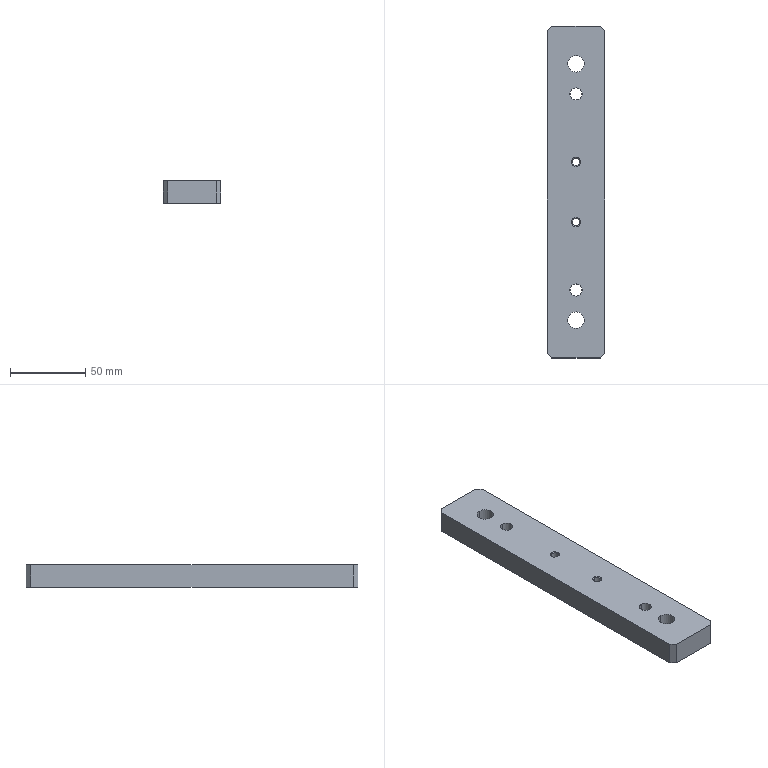Component | SolidWorks | DirectPressureVerticalSeal-1_TransitionPlate-1 | 1 solid | 30 faces | box 38 x 220 x 15 mm | volume 120177 mm3 | cylinder 12 | plane 10 | cone 8 | commonest cylinder face diameters 5 x4 8 x4 11 x4
build123d program:
from build123d import *

# Parameters (mm, degrees)
BOSS_EXTRUDE1_DEPTH                                  = 15
F_11_0_11_DIAMETER_HOLE1_D                           = 11
CONICAL_COUNTERSUNK_HOLE_1_FOR_M6_FLAT_H_D           = 8
CONICAL_COUNTERSUNK_HOLE_1_FOR_M6_FLAT_H_CSINK_D     = 8.05
CONICAL_COUNTERSUNK_HOLE_1_FOR_M6_FLAT_H_CSINK_ANGLE = 90
F_5_0_5_DIAMETER_HOLE1_D                             = 5
F_5_0_5_DIAMETER_HOLE1_CSINK_D                       = 6.05
F_5_0_5_DIAMETER_HOLE1_CSINK_ANGLE                   = 90


with BuildPart() as part:
    # Sketch1 → Boss-Extrude1 (new body)
    with BuildSketch(Plane.XY.offset(7.5)):
        Polygon((-110, 16), (-110, -16), (-107, -19), (107, -19), (110, -16), (110, 16), (107, 19), (-107, 19), align=None)
    extrude(amount=-BOSS_EXTRUDE1_DEPTH)

    # 11.0 _11_ Diameter Hole1 (through all)
    with Locations(Plane(origin=(0, 0, -7.5), x_dir=(-1, 0, 0), z_dir=(0, 0, -1))):
        with Locations((-85, 0), (85, 0)):
            Hole(F_11_0_11_DIAMETER_HOLE1_D / 2)

    # Conical Countersunk Hole 1 for M6 Flat H (through all)
    with Locations(Plane.XY.offset(7.5)):
        with Locations((65, 0), (-65, 0)):
            CounterSinkHole(CONICAL_COUNTERSUNK_HOLE_1_FOR_M6_FLAT_H_D / 2, CONICAL_COUNTERSUNK_HOLE_1_FOR_M6_FLAT_H_CSINK_D / 2, counter_sink_angle=CONICAL_COUNTERSUNK_HOLE_1_FOR_M6_FLAT_H_CSINK_ANGLE)

    # 5.0 _5_ Diameter Hole1 (through all)
    with Locations(Plane.XY.offset(7.5)):
        with Locations((20, 0), (-20, 0)):
            CounterSinkHole(F_5_0_5_DIAMETER_HOLE1_D / 2, F_5_0_5_DIAMETER_HOLE1_CSINK_D / 2, counter_sink_angle=F_5_0_5_DIAMETER_HOLE1_CSINK_ANGLE)


solid = part.part

# Placed as in the assembly
solid = solid.moved(Location((-298.746, 246.873, 246.554), (0, 0, 90)))
STEP:
#1=COLOUR_RGB('',0.7922,0.8196,0.9333);
#2=FILL_AREA_STYLE_COLOUR('',#1);
#3=FILL_AREA_STYLE('',(#2));
#4=SURFACE_STYLE_FILL_AREA(#3);
#5=SURFACE_SIDE_STYLE('',(#4));
#6=SURFACE_STYLE_USAGE(.BOTH.,#5);
#7=PRESENTATION_STYLE_ASSIGNMENT((#6));
#8=CARTESIAN_POINT('',(-11.762,9.03,9.981));
#9=VERTEX_POINT('',#8);
#10=CARTESIAN_POINT('',(-11.762,8.834,9.981));
#11=VERTEX_POINT('',#10);
#12=CARTESIAN_POINT('',(-11.762,8.932,9.981));
#13=DIRECTION('',(-0.,0.,1.));
#14=DIRECTION('',(0.,-1.,0.));
#15=AXIS2_PLACEMENT_3D('',#12,#13,#14);
#16=CIRCLE('',#15,0.09843);
#17=EDGE_CURVE('',#9,#11,#16,.T.);
#18=ORIENTED_EDGE('',*,*,#17,.F.);
#19=CARTESIAN_POINT('',(-11.762,9.051,10.002));
#20=VERTEX_POINT('',#19);
#21=CARTESIAN_POINT('',(-11.762,9.051,10.002));
#22=DIRECTION('',(0.,0.7071,0.7071));
#23=VECTOR('',#22,39.37);
#24=LINE('',#21,#23);
#25=EDGE_CURVE('',#9,#20,#24,.T.);
#26=ORIENTED_EDGE('',*,*,#25,.T.);
#27=CARTESIAN_POINT('',(-11.762,8.813,10.002));
#28=VERTEX_POINT('',#27);
#29=CARTESIAN_POINT('',(-11.762,8.932,10.002));
#30=DIRECTION('',(-0.,0.,1.));
#31=DIRECTION('',(0.,-1.,0.));
#32=AXIS2_PLACEMENT_3D('',#29,#30,#31);
#33=CIRCLE('',#32,0.1191);
#34=EDGE_CURVE('',#20,#28,#33,.T.);
#35=ORIENTED_EDGE('',*,*,#34,.T.);
#36=CARTESIAN_POINT('',(-11.762,8.813,10.002));
#37=DIRECTION('',(-0.,-0.7071,0.7071));
#38=VECTOR('',#37,39.37);
#39=LINE('',#36,#38);
#40=EDGE_CURVE('',#11,#28,#39,.T.);
#41=ORIENTED_EDGE('',*,*,#40,.F.);
#42=EDGE_LOOP('',(#18,#26,#35,#41));
#43=FACE_OUTER_BOUND('',#42,.T.);
#44=CARTESIAN_POINT('',(-11.762,8.932,10.002));
#45=DIRECTION('',(-0.,0.,1.));
#46=DIRECTION('',(0.,-1.,0.));
#47=AXIS2_PLACEMENT_3D('',#44,#45,#46);
#48=CONICAL_SURFACE('',#47,0.1191,0.7854);
#49=ADVANCED_FACE('',(#43),#48,.F.);
#50=CARTESIAN_POINT('',(-11.762,9.03,9.412));
#51=VERTEX_POINT('',#50);
#52=CARTESIAN_POINT('',(-11.762,8.834,9.412));
#53=VERTEX_POINT('',#52);
#54=CARTESIAN_POINT('',(-11.762,8.932,9.412));
#55=DIRECTION('',(-0.,0.,1.));
#56=DIRECTION('',(0.,-1.,0.));
#57=AXIS2_PLACEMENT_3D('',#54,#55,#56);
#58=CIRCLE('',#57,0.09843);
#59=EDGE_CURVE('',#51,#53,#58,.T.);
#60=ORIENTED_EDGE('',*,*,#59,.F.);
#61=CARTESIAN_POINT('',(-11.762,9.03,10.002));
#62=DIRECTION('',(-0.,0.,1.));
#63=VECTOR('',#62,39.37);
#64=LINE('',#61,#63);
#65=EDGE_CURVE('',#51,#9,#64,.T.);
#66=ORIENTED_EDGE('',*,*,#65,.T.);
#67=ORIENTED_EDGE('',*,*,#17,.T.);
#68=CARTESIAN_POINT('',(-11.762,8.834,10.002));
#69=DIRECTION('',(-0.,0.,1.));
#70=VECTOR('',#69,39.37);
#71=LINE('',#68,#70);
#72=EDGE_CURVE('',#53,#11,#71,.T.);
#73=ORIENTED_EDGE('',*,*,#72,.F.);
#74=EDGE_LOOP('',(#60,#66,#67,#73));
#75=FACE_OUTER_BOUND('',#74,.T.);
#76=CARTESIAN_POINT('',(-11.762,8.932,10.002));
#77=DIRECTION('',(-0.,0.,1.));
#78=DIRECTION('',(0.,-1.,0.));
#79=AXIS2_PLACEMENT_3D('',#76,#77,#78);
#80=CYLINDRICAL_SURFACE('',#79,0.09843);
#81=ADVANCED_FACE('',(#75),#80,.F.);
#82=CARTESIAN_POINT('',(-11.762,10.605,9.981));
#83=VERTEX_POINT('',#82);
#84=CARTESIAN_POINT('',(-11.762,10.408,9.981));
#85=VERTEX_POINT('',#84);
#86=CARTESIAN_POINT('',(-11.762,10.507,9.981));
#87=DIRECTION('',(-0.,0.,1.));
#88=DIRECTION('',(0.,-1.,0.));
#89=AXIS2_PLACEMENT_3D('',#86,#87,#88);
#90=CIRCLE('',#89,0.09843);
#91=EDGE_CURVE('',#83,#85,#90,.T.);
#92=ORIENTED_EDGE('',*,*,#91,.F.);
#93=CARTESIAN_POINT('',(-11.762,10.626,10.002));
#94=VERTEX_POINT('',#93);
#95=CARTESIAN_POINT('',(-11.762,10.626,10.002));
#96=DIRECTION('',(0.,0.7071,0.7071));
#97=VECTOR('',#96,39.37);
#98=LINE('',#95,#97);
#99=EDGE_CURVE('',#83,#94,#98,.T.);
#100=ORIENTED_EDGE('',*,*,#99,.T.);
#101=CARTESIAN_POINT('',(-11.762,10.388,10.002));
#102=VERTEX_POINT('',#101);
#103=CARTESIAN_POINT('',(-11.762,10.507,10.002));
#104=DIRECTION('',(-0.,0.,1.));
#105=DIRECTION('',(0.,-1.,0.));
#106=AXIS2_PLACEMENT_3D('',#103,#104,#105);
#107=CIRCLE('',#106,0.1191);
#108=EDGE_CURVE('',#94,#102,#107,.T.);
#109=ORIENTED_EDGE('',*,*,#108,.T.);
#110=CARTESIAN_POINT('',(-11.762,10.388,10.002));
#111=DIRECTION('',(-0.,-0.7071,0.7071));
#112=VECTOR('',#111,39.37);
#113=LINE('',#110,#112);
#114=EDGE_CURVE('',#85,#102,#113,.T.);
#115=ORIENTED_EDGE('',*,*,#114,.F.);
#116=EDGE_LOOP('',(#92,#100,#109,#115));
#117=FACE_OUTER_BOUND('',#116,.T.);
#118=CARTESIAN_POINT('',(-11.762,10.507,10.002));
#119=DIRECTION('',(-0.,0.,1.));
#120=DIRECTION('',(0.,-1.,0.));
#121=AXIS2_PLACEMENT_3D('',#118,#119,#120);
#122=CONICAL_SURFACE('',#121,0.1191,0.7854);
#123=ADVANCED_FACE('',(#117),#122,.F.);
#124=CARTESIAN_POINT('',(-11.762,10.605,9.412));
#125=VERTEX_POINT('',#124);
#126=CARTESIAN_POINT('',(-11.762,10.408,9.412));
#127=VERTEX_POINT('',#126);
#128=CARTESIAN_POINT('',(-11.762,10.507,9.412));
#129=DIRECTION('',(-0.,0.,1.));
#130=DIRECTION('',(0.,-1.,0.));
#131=AXIS2_PLACEMENT_3D('',#128,#129,#130);
#132=CIRCLE('',#131,0.09843);
#133=EDGE_CURVE('',#125,#127,#132,.T.);
#134=ORIENTED_EDGE('',*,*,#133,.F.);
#135=CARTESIAN_POINT('',(-11.762,10.605,10.002));
#136=DIRECTION('',(-0.,0.,1.));
#137=VECTOR('',#136,39.37);
#138=LINE('',#135,#137);
#139=EDGE_CURVE('',#125,#83,#138,.T.);
#140=ORIENTED_EDGE('',*,*,#139,.T.);
#141=ORIENTED_EDGE('',*,*,#91,.T.);
#142=CARTESIAN_POINT('',(-11.762,10.408,10.002));
#143=DIRECTION('',(-0.,0.,1.));
#144=VECTOR('',#143,39.37);
#145=LINE('',#142,#144);
#146=EDGE_CURVE('',#127,#85,#145,.T.);
#147=ORIENTED_EDGE('',*,*,#146,.F.);
#148=EDGE_LOOP('',(#134,#140,#141,#147));
#149=FACE_OUTER_BOUND('',#148,.T.);
#150=CARTESIAN_POINT('',(-11.762,10.507,10.002));
#151=DIRECTION('',(-0.,0.,1.));
#152=DIRECTION('',(0.,-1.,0.));
#153=AXIS2_PLACEMENT_3D('',#150,#151,#152);
#154=CYLINDRICAL_SURFACE('',#153,0.09843);
#155=ADVANCED_FACE('',(#149),#154,.F.);
#156=CARTESIAN_POINT('',(-11.762,7.318,10.001));
#157=VERTEX_POINT('',#156);
#158=CARTESIAN_POINT('',(-11.762,7.003,10.001));
#159=VERTEX_POINT('',#158);
#160=CARTESIAN_POINT('',(-11.762,7.16,10.001));
#161=DIRECTION('',(-0.,0.,1.));
#162=DIRECTION('',(0.,-1.,0.));
#163=AXIS2_PLACEMENT_3D('',#160,#161,#162);
#164=CIRCLE('',#163,0.1575);
#165=EDGE_CURVE('',#157,#159,#164,.T.);
#166=ORIENTED_EDGE('',*,*,#165,.F.);
#167=CARTESIAN_POINT('',(-11.762,7.319,10.002));
#168=VERTEX_POINT('',#167);
#169=CARTESIAN_POINT('',(-11.762,7.319,10.002));
#170=DIRECTION('',(0.,0.7071,0.7071));
#171=VECTOR('',#170,39.37);
#172=LINE('',#169,#171);
#173=EDGE_CURVE('',#157,#168,#172,.T.);
#174=ORIENTED_EDGE('',*,*,#173,.T.);
#175=CARTESIAN_POINT('',(-11.762,7.002,10.002));
#176=VERTEX_POINT('',#175);
#177=CARTESIAN_POINT('',(-11.762,7.16,10.002));
#178=DIRECTION('',(-0.,0.,1.));
#179=DIRECTION('',(0.,-1.,0.));
#180=AXIS2_PLACEMENT_3D('',#177,#178,#179);
#181=CIRCLE('',#180,0.1585);
#182=EDGE_CURVE('',#168,#176,#181,.T.);
#183=ORIENTED_EDGE('',*,*,#182,.T.);
#184=CARTESIAN_POINT('',(-11.762,7.002,10.002));
#185=DIRECTION('',(-0.,-0.7071,0.7071));
#186=VECTOR('',#185,39.37);
#187=LINE('',#184,#186);
#188=EDGE_CURVE('',#159,#176,#187,.T.);
#189=ORIENTED_EDGE('',*,*,#188,.F.);
#190=EDGE_LOOP('',(#166,#174,#183,#189));
#191=FACE_OUTER_BOUND('',#190,.T.);
#192=CARTESIAN_POINT('',(-11.762,7.16,10.002));
#193=DIRECTION('',(-0.,0.,1.));
#194=DIRECTION('',(0.,-1.,0.));
#195=AXIS2_PLACEMENT_3D('',#192,#193,#194);
#196=CONICAL_SURFACE('',#195,0.1585,0.7854);
#197=ADVANCED_FACE('',(#191),#196,.F.);
#198=CARTESIAN_POINT('',(-11.762,7.318,9.412));
#199=VERTEX_POINT('',#198);
#200=CARTESIAN_POINT('',(-11.762,7.003,9.412));
#201=VERTEX_POINT('',#200);
#202=CARTESIAN_POINT('',(-11.762,7.16,9.412));
#203=DIRECTION('',(-0.,0.,1.));
#204=DIRECTION('',(0.,-1.,0.));
#205=AXIS2_PLACEMENT_3D('',#202,#203,#204);
#206=CIRCLE('',#205,0.1575);
#207=EDGE_CURVE('',#199,#201,#206,.T.);
#208=ORIENTED_EDGE('',*,*,#207,.F.);
#209=CARTESIAN_POINT('',(-11.762,7.318,10.002));
#210=DIRECTION('',(-0.,0.,1.));
#211=VECTOR('',#210,39.37);
#212=LINE('',#209,#211);
#213=EDGE_CURVE('',#199,#157,#212,.T.);
#214=ORIENTED_EDGE('',*,*,#213,.T.);
#215=ORIENTED_EDGE('',*,*,#165,.T.);
#216=CARTESIAN_POINT('',(-11.762,7.003,10.002));
#217=DIRECTION('',(-0.,0.,1.));
#218=VECTOR('',#217,39.37);
#219=LINE('',#216,#218);
#220=EDGE_CURVE('',#201,#159,#219,.T.);
#221=ORIENTED_EDGE('',*,*,#220,.F.);
#222=EDGE_LOOP('',(#208,#214,#215,#221));
#223=FACE_OUTER_BOUND('',#222,.T.);
#224=CARTESIAN_POINT('',(-11.762,7.16,10.002));
#225=DIRECTION('',(-0.,0.,1.));
#226=DIRECTION('',(0.,-1.,0.));
#227=AXIS2_PLACEMENT_3D('',#224,#225,#226);
#228=CYLINDRICAL_SURFACE('',#227,0.1575);
#229=ADVANCED_FACE('',(#223),#228,.F.);
#230=CARTESIAN_POINT('',(-11.762,12.436,10.001));
#231=VERTEX_POINT('',#230);
#232=CARTESIAN_POINT('',(-11.762,12.121,10.001));
#233=VERTEX_POINT('',#232);
#234=CARTESIAN_POINT('',(-11.762,12.278,10.001));
#235=DIRECTION('',(-0.,0.,1.));
#236=DIRECTION('',(0.,-1.,0.));
#237=AXIS2_PLACEMENT_3D('',#234,#235,#236);
#238=CIRCLE('',#237,0.1575);
#239=EDGE_CURVE('',#231,#233,#238,.T.);
#240=ORIENTED_EDGE('',*,*,#239,.F.);
#241=CARTESIAN_POINT('',(-11.762,12.437,10.002));
#242=VERTEX_POINT('',#241);
#243=CARTESIAN_POINT('',(-11.762,12.437,10.002));
#244=DIRECTION('',(0.,0.7071,0.7071));
#245=VECTOR('',#244,39.37);
#246=LINE('',#243,#245);
#247=EDGE_CURVE('',#231,#242,#246,.T.);
#248=ORIENTED_EDGE('',*,*,#247,.T.);
#249=CARTESIAN_POINT('',(-11.762,12.12,10.002));
#250=VERTEX_POINT('',#249);
#251=CARTESIAN_POINT('',(-11.762,12.278,10.002));
#252=DIRECTION('',(-0.,0.,1.));
#253=DIRECTION('',(0.,-1.,0.));
#254=AXIS2_PLACEMENT_3D('',#251,#252,#253);
#255=CIRCLE('',#254,0.1585);
#256=EDGE_CURVE('',#242,#250,#255,.T.);
#257=ORIENTED_EDGE('',*,*,#256,.T.);
#258=CARTESIAN_POINT('',(-11.762,12.12,10.002));
#259=DIRECTION('',(-0.,-0.7071,0.7071));
#260=VECTOR('',#259,39.37);
#261=LINE('',#258,#260);
#262=EDGE_CURVE('',#233,#250,#261,.T.);
#263=ORIENTED_EDGE('',*,*,#262,.F.);
#264=EDGE_LOOP('',(#240,#248,#257,#263));
#265=FACE_OUTER_BOUND('',#264,.T.);
#266=CARTESIAN_POINT('',(-11.762,12.278,10.002));
#267=DIRECTION('',(-0.,0.,1.));
#268=DIRECTION('',(0.,-1.,0.));
#269=AXIS2_PLACEMENT_3D('',#266,#267,#268);
#270=CONICAL_SURFACE('',#269,0.1585,0.7854);
#271=ADVANCED_FACE('',(#265),#270,.F.);
#272=CARTESIAN_POINT('',(-11.762,12.436,9.412));
#273=VERTEX_POINT('',#272);
#274=CARTESIAN_POINT('',(-11.762,12.121,9.412));
#275=VERTEX_POINT('',#274);
#276=CARTESIAN_POINT('',(-11.762,12.278,9.412));
#277=DIRECTION('',(-0.,0.,1.));
#278=DIRECTION('',(0.,-1.,0.));
#279=AXIS2_PLACEMENT_3D('',#276,#277,#278);
#280=CIRCLE('',#279,0.1575);
#281=EDGE_CURVE('',#273,#275,#280,.T.);
#282=ORIENTED_EDGE('',*,*,#281,.F.);
#283=CARTESIAN_POINT('',(-11.762,12.436,10.002));
#284=DIRECTION('',(-0.,0.,1.));
#285=VECTOR('',#284,39.37);
#286=LINE('',#283,#285);
#287=EDGE_CURVE('',#273,#231,#286,.T.);
#288=ORIENTED_EDGE('',*,*,#287,.T.);
#289=ORIENTED_EDGE('',*,*,#239,.T.);
#290=CARTESIAN_POINT('',(-11.762,12.121,10.002));
#291=DIRECTION('',(-0.,0.,1.));
#292=VECTOR('',#291,39.37);
#293=LINE('',#290,#292);
#294=EDGE_CURVE('',#275,#233,#293,.T.);
#295=ORIENTED_EDGE('',*,*,#294,.F.);
#296=EDGE_LOOP('',(#282,#288,#289,#295));
#297=FACE_OUTER_BOUND('',#296,.T.);
#298=CARTESIAN_POINT('',(-11.762,12.278,10.002));
#299=DIRECTION('',(-0.,0.,1.));
#300=DIRECTION('',(0.,-1.,0.));
#301=AXIS2_PLACEMENT_3D('',#298,#299,#300);
#302=CYLINDRICAL_SURFACE('',#301,0.1575);
#303=ADVANCED_FACE('',(#297),#302,.F.);
#304=CARTESIAN_POINT('',(-11.762,6.156,10.002));
#305=VERTEX_POINT('',#304);
#306=CARTESIAN_POINT('',(-11.762,6.59,10.002));
#307=VERTEX_POINT('',#306);
#308=CARTESIAN_POINT('',(-11.762,6.373,10.002));
#309=DIRECTION('',(0.,-0.,-1.));
#310=DIRECTION('',(0.,1.,0.));
#311=AXIS2_PLACEMENT_3D('',#308,#309,#310);
#312=CIRCLE('',#311,0.2165);
#313=EDGE_CURVE('',#305,#307,#312,.T.);
#314=ORIENTED_EDGE('',*,*,#313,.F.);
#315=CARTESIAN_POINT('',(-11.762,6.156,9.412));
#316=VERTEX_POINT('',#315);
#317=CARTESIAN_POINT('',(-11.762,6.156,9.412));
#318=DIRECTION('',(0.,-0.,-1.));
#319=VECTOR('',#318,39.37);
#320=LINE('',#317,#319);
#321=EDGE_CURVE('',#305,#316,#320,.T.);
#322=ORIENTED_EDGE('',*,*,#321,.T.);
#323=CARTESIAN_POINT('',(-11.762,6.59,9.412));
#324=VERTEX_POINT('',#323);
#325=CARTESIAN_POINT('',(-11.762,6.373,9.412));
#326=DIRECTION('',(0.,-0.,-1.));
#327=DIRECTION('',(0.,1.,0.));
#328=AXIS2_PLACEMENT_3D('',#325,#326,#327);
#329=CIRCLE('',#328,0.2165);
#330=EDGE_CURVE('',#316,#324,#329,.T.);
#331=ORIENTED_EDGE('',*,*,#330,.T.);
#332=CARTESIAN_POINT('',(-11.762,6.59,9.412));
#333=DIRECTION('',(0.,-0.,-1.));
#334=VECTOR('',#333,39.37);
#335=LINE('',#332,#334);
#336=EDGE_CURVE('',#307,#324,#335,.T.);
#337=ORIENTED_EDGE('',*,*,#336,.F.);
#338=EDGE_LOOP('',(#314,#322,#331,#337));
#339=FACE_OUTER_BOUND('',#338,.T.);
#340=CARTESIAN_POINT('',(-11.762,6.373,9.412));
#341=DIRECTION('',(0.,-0.,-1.));
#342=DIRECTION('',(0.,1.,0.));
#343=AXIS2_PLACEMENT_3D('',#340,#341,#342);
#344=CYLINDRICAL_SURFACE('',#343,0.2165);
#345=ADVANCED_FACE('',(#339),#344,.F.);
#346=CARTESIAN_POINT('',(-11.762,12.849,10.002));
#347=VERTEX_POINT('',#346);
#348=CARTESIAN_POINT('',(-11.762,13.282,10.002));
#349=VERTEX_POINT('',#348);
#350=CARTESIAN_POINT('',(-11.762,13.066,10.002));
#351=DIRECTION('',(0.,-0.,-1.));
#352=DIRECTION('',(0.,1.,0.));
#353=AXIS2_PLACEMENT_3D('',#350,#351,#352);
#354=CIRCLE('',#353,0.2165);
#355=EDGE_CURVE('',#347,#349,#354,.T.);
#356=ORIENTED_EDGE('',*,*,#355,.F.);
#357=CARTESIAN_POINT('',(-11.762,12.849,9.412));
#358=VERTEX_POINT('',#357);
#359=CARTESIAN_POINT('',(-11.762,12.849,9.412));
#360=DIRECTION('',(0.,-0.,-1.));
#361=VECTOR('',#360,39.37);
#362=LINE('',#359,#361);
#363=EDGE_CURVE('',#347,#358,#362,.T.);
#364=ORIENTED_EDGE('',*,*,#363,.T.);
#365=CARTESIAN_POINT('',(-11.762,13.282,9.412));
#366=VERTEX_POINT('',#365);
#367=CARTESIAN_POINT('',(-11.762,13.066,9.412));
#368=DIRECTION('',(0.,-0.,-1.));
#369=DIRECTION('',(0.,1.,0.));
#370=AXIS2_PLACEMENT_3D('',#367,#368,#369);
#371=CIRCLE('',#370,0.2165);
#372=EDGE_CURVE('',#358,#366,#371,.T.);
#373=ORIENTED_EDGE('',*,*,#372,.T.);
#374=CARTESIAN_POINT('',(-11.762,13.282,9.412));
#375=DIRECTION('',(0.,-0.,-1.));
#376=VECTOR('',#375,39.37);
#377=LINE('',#374,#376);
#378=EDGE_CURVE('',#349,#366,#377,.T.);
#379=ORIENTED_EDGE('',*,*,#378,.F.);
#380=EDGE_LOOP('',(#356,#364,#373,#379));
#381=FACE_OUTER_BOUND('',#380,.T.);
#382=CARTESIAN_POINT('',(-11.762,13.066,9.412));
#383=DIRECTION('',(0.,-0.,-1.));
#384=DIRECTION('',(0.,1.,0.));
#385=AXIS2_PLACEMENT_3D('',#382,#383,#384);
#386=CYLINDRICAL_SURFACE('',#385,0.2165);
#387=ADVANCED_FACE('',(#381),#386,.F.);
#388=CARTESIAN_POINT('',(-11.014,13.932,10.002));
#389=VERTEX_POINT('',#388);
#390=CARTESIAN_POINT('',(-11.132,14.05,10.002));
#391=VERTEX_POINT('',#390);
#392=CARTESIAN_POINT('',(-11.014,13.932,10.002));
#393=DIRECTION('',(-0.7071,0.7071,-0.));
#394=VECTOR('',#393,39.37);
#395=LINE('',#392,#394);
#396=EDGE_CURVE('',#389,#391,#395,.T.);
#397=ORIENTED_EDGE('',*,*,#396,.F.);
#398=CARTESIAN_POINT('',(-11.014,13.932,9.412));
#399=VERTEX_POINT('',#398);
#400=CARTESIAN_POINT('',(-11.014,13.932,9.412));
#401=DIRECTION('',(-0.,0.,1.));
#402=VECTOR('',#401,39.37);
#403=LINE('',#400,#402);
#404=EDGE_CURVE('',#399,#389,#403,.T.);
#405=ORIENTED_EDGE('',*,*,#404,.F.);
#406=CARTESIAN_POINT('',(-11.132,14.05,9.412));
#407=VERTEX_POINT('',#406);
#408=CARTESIAN_POINT('',(-11.014,13.932,9.412));
#409=DIRECTION('',(-0.7071,0.7071,-0.));
#410=VECTOR('',#409,39.37);
#411=LINE('',#408,#410);
#412=EDGE_CURVE('',#399,#407,#411,.T.);
#413=ORIENTED_EDGE('',*,*,#412,.T.);
#414=CARTESIAN_POINT('',(-11.132,14.05,9.412));
#415=DIRECTION('',(-0.,0.,1.));
#416=VECTOR('',#415,39.37);
#417=LINE('',#414,#416);
#418=EDGE_CURVE('',#407,#391,#417,.T.);
#419=ORIENTED_EDGE('',*,*,#418,.T.);
#420=EDGE_LOOP('',(#397,#405,#413,#419));
#421=FACE_OUTER_BOUND('',#420,.T.);
#422=CARTESIAN_POINT('',(-11.014,13.932,9.412));
#423=DIRECTION('',(0.7071,0.7071,0.));
#424=DIRECTION('',(-0.7071,0.7071,-0.));
#425=AXIS2_PLACEMENT_3D('',#422,#423,#424);
#426=PLANE('',#425);
#427=ADVANCED_FACE('',(#421),#426,.T.);
#428=CARTESIAN_POINT('',(-11.014,5.507,10.002));
#429=VERTEX_POINT('',#428);
#430=CARTESIAN_POINT('',(-11.014,5.507,10.002));
#431=DIRECTION('',(0.,1.,-0.));
#432=VECTOR('',#431,39.37);
#433=LINE('',#430,#432);
#434=EDGE_CURVE('',#429,#389,#433,.T.);
#435=ORIENTED_EDGE('',*,*,#434,.F.);
#436=CARTESIAN_POINT('',(-11.014,5.507,9.412));
#437=VERTEX_POINT('',#436);
#438=CARTESIAN_POINT('',(-11.014,5.507,9.412));
#439=DIRECTION('',(-0.,0.,1.));
#440=VECTOR('',#439,39.37);
#441=LINE('',#438,#440);
#442=EDGE_CURVE('',#437,#429,#441,.T.);
#443=ORIENTED_EDGE('',*,*,#442,.F.);
#444=CARTESIAN_POINT('',(-11.014,5.507,9.412));
#445=DIRECTION('',(0.,1.,-0.));
#446=VECTOR('',#445,39.37);
#447=LINE('',#444,#446);
#448=EDGE_CURVE('',#437,#399,#447,.T.);
#449=ORIENTED_EDGE('',*,*,#448,.T.);
#450=ORIENTED_EDGE('',*,*,#404,.T.);
#451=EDGE_LOOP('',(#435,#443,#449,#450));
#452=FACE_OUTER_BOUND('',#451,.T.);
#453=CARTESIAN_POINT('',(-11.014,5.507,9.412));
#454=DIRECTION('',(1.,-0.,0.));
#455=DIRECTION('',(-0.,0.,1.));
#456=AXIS2_PLACEMENT_3D('',#453,#454,#455);
#457=PLANE('',#456);
#458=ADVANCED_FACE('',(#452),#457,.T.);
#459=CARTESIAN_POINT('',(-11.132,5.389,10.002));
#460=VERTEX_POINT('',#459);
#461=CARTESIAN_POINT('',(-11.132,5.389,10.002));
#462=DIRECTION('',(0.7071,0.7071,0.));
#463=VECTOR('',#462,39.37);
#464=LINE('',#461,#463);
#465=EDGE_CURVE('',#460,#429,#464,.T.);
#466=ORIENTED_EDGE('',*,*,#465,.F.);
#467=CARTESIAN_POINT('',(-11.132,5.389,9.412));
#468=VERTEX_POINT('',#467);
#469=CARTESIAN_POINT('',(-11.132,5.389,9.412));
#470=DIRECTION('',(-0.,0.,1.));
#471=VECTOR('',#470,39.37);
#472=LINE('',#469,#471);
#473=EDGE_CURVE('',#468,#460,#472,.T.);
#474=ORIENTED_EDGE('',*,*,#473,.F.);
#475=CARTESIAN_POINT('',(-11.132,5.389,9.412));
#476=DIRECTION('',(0.7071,0.7071,0.));
#477=VECTOR('',#476,39.37);
#478=LINE('',#475,#477);
#479=EDGE_CURVE('',#468,#437,#478,.T.);
#480=ORIENTED_EDGE('',*,*,#479,.T.);
#481=ORIENTED_EDGE('',*,*,#442,.T.);
#482=EDGE_LOOP('',(#466,#474,#480,#481));
#483=FACE_OUTER_BOUND('',#482,.T.);
#484=CARTESIAN_POINT('',(-11.132,5.389,9.412));
#485=DIRECTION('',(0.7071,-0.7071,0.));
#486=DIRECTION('',(0.7071,0.7071,0.));
#487=AXIS2_PLACEMENT_3D('',#484,#485,#486);
#488=PLANE('',#487);
#489=ADVANCED_FACE('',(#483),#488,.T.);
#490=CARTESIAN_POINT('',(-12.392,5.389,10.002));
#491=VERTEX_POINT('',#490);
#492=CARTESIAN_POINT('',(-12.392,5.389,10.002));
#493=DIRECTION('',(1.,-0.,0.));
#494=VECTOR('',#493,39.37);
#495=LINE('',#492,#494);
#496=EDGE_CURVE('',#491,#460,#495,.T.);
#497=ORIENTED_EDGE('',*,*,#496,.F.);
#498=CARTESIAN_POINT('',(-12.392,5.389,9.412));
#499=VERTEX_POINT('',#498);
#500=CARTESIAN_POINT('',(-12.392,5.389,9.412));
#501=DIRECTION('',(-0.,0.,1.));
#502=VECTOR('',#501,39.37);
#503=LINE('',#500,#502);
#504=EDGE_CURVE('',#499,#491,#503,.T.);
#505=ORIENTED_EDGE('',*,*,#504,.F.);
#506=CARTESIAN_POINT('',(-12.392,5.389,9.412));
#507=DIRECTION('',(1.,-0.,0.));
#508=VECTOR('',#507,39.37);
#509=LINE('',#506,#508);
#510=EDGE_CURVE('',#499,#468,#509,.T.);
#511=ORIENTED_EDGE('',*,*,#510,.T.);
#512=ORIENTED_EDGE('',*,*,#473,.T.);
#513=EDGE_LOOP('',(#497,#505,#511,#512));
#514=FACE_OUTER_BOUND('',#513,.T.);
#515=CARTESIAN_POINT('',(-12.392,5.389,9.412));
#516=DIRECTION('',(-0.,-1.,0.));
#517=DIRECTION('',(0.,-0.,-1.));
#518=AXIS2_PLACEMENT_3D('',#515,#516,#517);
#519=PLANE('',#518);
#520=ADVANCED_FACE('',(#514),#519,.T.);
#521=CARTESIAN_POINT('',(-12.51,5.507,10.002));
#522=VERTEX_POINT('',#521);
#523=CARTESIAN_POINT('',(-12.51,5.507,10.002));
#524=DIRECTION('',(0.7071,-0.7071,0.));
#525=VECTOR('',#524,39.37);
#526=LINE('',#523,#525);
#527=EDGE_CURVE('',#522,#491,#526,.T.);
#528=ORIENTED_EDGE('',*,*,#527,.F.);
#529=CARTESIAN_POINT('',(-12.51,5.507,9.412));
#530=VERTEX_POINT('',#529);
#531=CARTESIAN_POINT('',(-12.51,5.507,9.412));
#532=DIRECTION('',(-0.,0.,1.));
#533=VECTOR('',#532,39.37);
#534=LINE('',#531,#533);
#535=EDGE_CURVE('',#530,#522,#534,.T.);
#536=ORIENTED_EDGE('',*,*,#535,.F.);
#537=CARTESIAN_POINT('',(-12.51,5.507,9.412));
#538=DIRECTION('',(0.7071,-0.7071,0.));
#539=VECTOR('',#538,39.37);
#540=LINE('',#537,#539);
#541=EDGE_CURVE('',#530,#499,#540,.T.);
#542=ORIENTED_EDGE('',*,*,#541,.T.);
#543=ORIENTED_EDGE('',*,*,#504,.T.);
#544=EDGE_LOOP('',(#528,#536,#542,#543));
#545=FACE_OUTER_BOUND('',#544,.T.);
#546=CARTESIAN_POINT('',(-12.51,5.507,9.412));
#547=DIRECTION('',(-0.7071,-0.7071,-0.));
#548=DIRECTION('',(0.7071,-0.7071,0.));
#549=AXIS2_PLACEMENT_3D('',#546,#547,#548);
#550=PLANE('',#549);
#551=ADVANCED_FACE('',(#545),#550,.T.);
#552=CARTESIAN_POINT('',(-12.51,13.932,10.002));
#553=VERTEX_POINT('',#552);
#554=CARTESIAN_POINT('',(-12.51,13.932,10.002));
#555=DIRECTION('',(-0.,-1.,0.));
#556=VECTOR('',#555,39.37);
#557=LINE('',#554,#556);
#558=EDGE_CURVE('',#553,#522,#557,.T.);
#559=ORIENTED_EDGE('',*,*,#558,.F.);
#560=CARTESIAN_POINT('',(-12.51,13.932,9.412));
#561=VERTEX_POINT('',#560);
#562=CARTESIAN_POINT('',(-12.51,13.932,9.412));
#563=DIRECTION('',(-0.,0.,1.));
#564=VECTOR('',#563,39.37);
#565=LINE('',#562,#564);
#566=EDGE_CURVE('',#561,#553,#565,.T.);
#567=ORIENTED_EDGE('',*,*,#566,.F.);
#568=CARTESIAN_POINT('',(-12.51,13.932,9.412));
#569=DIRECTION('',(-0.,-1.,0.));
#570=VECTOR('',#569,39.37);
#571=LINE('',#568,#570);
#572=EDGE_CURVE('',#561,#530,#571,.T.);
#573=ORIENTED_EDGE('',*,*,#572,.T.);
#574=ORIENTED_EDGE('',*,*,#535,.T.);
#575=EDGE_LOOP('',(#559,#567,#573,#574));
#576=FACE_OUTER_BOUND('',#575,.T.);
#577=CARTESIAN_POINT('',(-12.51,13.932,9.412));
#578=DIRECTION('',(-1.,0.,-0.));
#579=DIRECTION('',(0.,-0.,-1.));
#580=AXIS2_PLACEMENT_3D('',#577,#578,#579);
#581=PLANE('',#580);
#582=ADVANCED_FACE('',(#576),#581,.T.);
#583=CARTESIAN_POINT('',(-12.392,14.05,10.002));
#584=VERTEX_POINT('',#583);
#585=CARTESIAN_POINT('',(-12.392,14.05,10.002));
#586=DIRECTION('',(-0.7071,-0.7071,-0.));
#587=VECTOR('',#586,39.37);
#588=LINE('',#585,#587);
#589=EDGE_CURVE('',#584,#553,#588,.T.);
#590=ORIENTED_EDGE('',*,*,#589,.F.);
#591=CARTESIAN_POINT('',(-12.392,14.05,9.412));
#592=VERTEX_POINT('',#591);
#593=CARTESIAN_POINT('',(-12.392,14.05,9.412));
#594=DIRECTION('',(-0.,0.,1.));
#595=VECTOR('',#594,39.37);
#596=LINE('',#593,#595);
#597=EDGE_CURVE('',#592,#584,#596,.T.);
#598=ORIENTED_EDGE('',*,*,#597,.F.);
#599=CARTESIAN_POINT('',(-12.392,14.05,9.412));
#600=DIRECTION('',(-0.7071,-0.7071,-0.));
#601=VECTOR('',#600,39.37);
#602=LINE('',#599,#601);
#603=EDGE_CURVE('',#592,#561,#602,.T.);
#604=ORIENTED_EDGE('',*,*,#603,.T.);
#605=ORIENTED_EDGE('',*,*,#566,.T.);
#606=EDGE_LOOP('',(#590,#598,#604,#605));
#607=FACE_OUTER_BOUND('',#606,.T.);
#608=CARTESIAN_POINT('',(-12.392,14.05,9.412));
#609=DIRECTION('',(-0.7071,0.7071,-0.));
#610=DIRECTION('',(-0.7071,-0.7071,-0.));
#611=AXIS2_PLACEMENT_3D('',#608,#609,#610);
#612=PLANE('',#611);
#613=ADVANCED_FACE('',(#607),#612,.T.);
#614=CARTESIAN_POINT('',(-11.132,14.05,10.002));
#615=DIRECTION('',(-1.,0.,-0.));
#616=VECTOR('',#615,39.37);
#617=LINE('',#614,#616);
#618=EDGE_CURVE('',#391,#584,#617,.T.);
#619=ORIENTED_EDGE('',*,*,#618,.F.);
#620=ORIENTED_EDGE('',*,*,#418,.F.);
#621=CARTESIAN_POINT('',(-11.132,14.05,9.412));
#622=DIRECTION('',(-1.,0.,-0.));
#623=VECTOR('',#622,39.37);
#624=LINE('',#621,#623);
#625=EDGE_CURVE('',#407,#592,#624,.T.);
#626=ORIENTED_EDGE('',*,*,#625,.T.);
#627=ORIENTED_EDGE('',*,*,#597,.T.);
#628=EDGE_LOOP('',(#619,#620,#626,#627));
#629=FACE_OUTER_BOUND('',#628,.T.);
#630=CARTESIAN_POINT('',(-11.132,14.05,9.412));
#631=DIRECTION('',(0.,1.,-0.));
#632=DIRECTION('',(-1.,0.,-0.));
#633=AXIS2_PLACEMENT_3D('',#630,#631,#632);
#634=PLANE('',#633);
#635=ADVANCED_FACE('',(#629),#634,.T.);
#636=CARTESIAN_POINT('',(-11.762,8.932,9.412));
#637=DIRECTION('',(-0.,0.,1.));
#638=DIRECTION('',(0.,-1.,0.));
#639=AXIS2_PLACEMENT_3D('',#636,#637,#638);
#640=CIRCLE('',#639,0.09843);
#641=EDGE_CURVE('',#53,#51,#640,.T.);
#642=ORIENTED_EDGE('',*,*,#641,.T.);
#643=ORIENTED_EDGE('',*,*,#59,.T.);
#644=EDGE_LOOP('',(#642,#643));
#645=FACE_BOUND('',#644,.T.);
#646=CARTESIAN_POINT('',(-11.762,10.507,9.412));
#647=DIRECTION('',(-0.,0.,1.));
#648=DIRECTION('',(0.,-1.,0.));
#649=AXIS2_PLACEMENT_3D('',#646,#647,#648);
#650=CIRCLE('',#649,0.09843);
#651=EDGE_CURVE('',#127,#125,#650,.T.);
#652=ORIENTED_EDGE('',*,*,#651,.T.);
#653=ORIENTED_EDGE('',*,*,#133,.T.);
#654=EDGE_LOOP('',(#652,#653));
#655=FACE_BOUND('',#654,.T.);
#656=CARTESIAN_POINT('',(-11.762,7.16,9.412));
#657=DIRECTION('',(-0.,0.,1.));
#658=DIRECTION('',(0.,-1.,0.));
#659=AXIS2_PLACEMENT_3D('',#656,#657,#658);
#660=CIRCLE('',#659,0.1575);
#661=EDGE_CURVE('',#201,#199,#660,.T.);
#662=ORIENTED_EDGE('',*,*,#661,.T.);
#663=ORIENTED_EDGE('',*,*,#207,.T.);
#664=EDGE_LOOP('',(#662,#663));
#665=FACE_BOUND('',#664,.T.);
#666=CARTESIAN_POINT('',(-11.762,12.278,9.412));
#667=DIRECTION('',(-0.,0.,1.));
#668=DIRECTION('',(0.,-1.,0.));
#669=AXIS2_PLACEMENT_3D('',#666,#667,#668);
#670=CIRCLE('',#669,0.1575);
#671=EDGE_CURVE('',#275,#273,#670,.T.);
#672=ORIENTED_EDGE('',*,*,#671,.T.);
#673=ORIENTED_EDGE('',*,*,#281,.T.);
#674=EDGE_LOOP('',(#672,#673));
#675=FACE_BOUND('',#674,.T.);
#676=CARTESIAN_POINT('',(-11.762,6.373,9.412));
#677=DIRECTION('',(0.,-0.,-1.));
#678=DIRECTION('',(0.,1.,0.));
#679=AXIS2_PLACEMENT_3D('',#676,#677,#678);
#680=CIRCLE('',#679,0.2165);
#681=EDGE_CURVE('',#324,#316,#680,.T.);
#682=ORIENTED_EDGE('',*,*,#681,.F.);
#683=ORIENTED_EDGE('',*,*,#330,.F.);
#684=EDGE_LOOP('',(#682,#683));
#685=FACE_BOUND('',#684,.T.);
#686=CARTESIAN_POINT('',(-11.762,13.066,9.412));
#687=DIRECTION('',(0.,-0.,-1.));
#688=DIRECTION('',(0.,1.,0.));
#689=AXIS2_PLACEMENT_3D('',#686,#687,#688);
#690=CIRCLE('',#689,0.2165);
#691=EDGE_CURVE('',#366,#358,#690,.T.);
#692=ORIENTED_EDGE('',*,*,#691,.F.);
#693=ORIENTED_EDGE('',*,*,#372,.F.);
#694=EDGE_LOOP('',(#692,#693));
#695=FACE_BOUND('',#694,.T.);
#696=ORIENTED_EDGE('',*,*,#412,.F.);
#697=ORIENTED_EDGE('',*,*,#448,.F.);
#698=ORIENTED_EDGE('',*,*,#479,.F.);
#699=ORIENTED_EDGE('',*,*,#510,.F.);
#700=ORIENTED_EDGE('',*,*,#541,.F.);
#701=ORIENTED_EDGE('',*,*,#572,.F.);
#702=ORIENTED_EDGE('',*,*,#603,.F.);
#703=ORIENTED_EDGE('',*,*,#625,.F.);
#704=EDGE_LOOP('',(#696,#697,#698,#699,#700,#701,#702,#703));
#705=FACE_OUTER_BOUND('',#704,.T.);
#706=CARTESIAN_POINT('',(-11.762,9.719,9.412));
#707=DIRECTION('',(-0.,0.,1.));
#708=DIRECTION('',(-0.,-1.,0.));
#709=AXIS2_PLACEMENT_3D('',#706,#707,#708);
#710=PLANE('',#709);
#711=ADVANCED_FACE('',(#645,#655,#665,#675,#685,#695,#705),#710,.F.);
#712=CARTESIAN_POINT('',(-11.762,8.932,10.002));
#713=DIRECTION('',(-0.,0.,1.));
#714=DIRECTION('',(0.,-1.,0.));
#715=AXIS2_PLACEMENT_3D('',#712,#713,#714);
#716=CIRCLE('',#715,0.1191);
#717=EDGE_CURVE('',#28,#20,#716,.T.);
#718=ORIENTED_EDGE('',*,*,#717,.F.);
#719=ORIENTED_EDGE('',*,*,#34,.F.);
#720=EDGE_LOOP('',(#718,#719));
#721=FACE_BOUND('',#720,.T.);
#722=CARTESIAN_POINT('',(-11.762,10.507,10.002));
#723=DIRECTION('',(-0.,0.,1.));
#724=DIRECTION('',(0.,-1.,0.));
#725=AXIS2_PLACEMENT_3D('',#722,#723,#724);
#726=CIRCLE('',#725,0.1191);
#727=EDGE_CURVE('',#102,#94,#726,.T.);
#728=ORIENTED_EDGE('',*,*,#727,.F.);
#729=ORIENTED_EDGE('',*,*,#108,.F.);
#730=EDGE_LOOP('',(#728,#729));
#731=FACE_BOUND('',#730,.T.);
#732=CARTESIAN_POINT('',(-11.762,7.16,10.002));
#733=DIRECTION('',(-0.,0.,1.));
#734=DIRECTION('',(0.,-1.,0.));
#735=AXIS2_PLACEMENT_3D('',#732,#733,#734);
#736=CIRCLE('',#735,0.1585);
#737=EDGE_CURVE('',#176,#168,#736,.T.);
#738=ORIENTED_EDGE('',*,*,#737,.F.);
#739=ORIENTED_EDGE('',*,*,#182,.F.);
#740=EDGE_LOOP('',(#738,#739));
#741=FACE_BOUND('',#740,.T.);
#742=CARTESIAN_POINT('',(-11.762,12.278,10.002));
#743=DIRECTION('',(-0.,0.,1.));
#744=DIRECTION('',(0.,-1.,0.));
#745=AXIS2_PLACEMENT_3D('',#742,#743,#744);
#746=CIRCLE('',#745,0.1585);
#747=EDGE_CURVE('',#250,#242,#746,.T.);
#748=ORIENTED_EDGE('',*,*,#747,.F.);
#749=ORIENTED_EDGE('',*,*,#256,.F.);
#750=EDGE_LOOP('',(#748,#749));
#751=FACE_BOUND('',#750,.T.);
#752=CARTESIAN_POINT('',(-11.762,6.373,10.002));
#753=DIRECTION('',(0.,-0.,-1.));
#754=DIRECTION('',(0.,1.,0.));
#755=AXIS2_PLACEMENT_3D('',#752,#753,#754);
#756=CIRCLE('',#755,0.2165);
#757=EDGE_CURVE('',#307,#305,#756,.T.);
#758=ORIENTED_EDGE('',*,*,#757,.T.);
#759=ORIENTED_EDGE('',*,*,#313,.T.);
#760=EDGE_LOOP('',(#758,#759));
#761=FACE_BOUND('',#760,.T.);
#762=CARTESIAN_POINT('',(-11.762,13.066,10.002));
#763=DIRECTION('',(0.,-0.,-1.));
#764=DIRECTION('',(0.,1.,0.));
#765=AXIS2_PLACEMENT_3D('',#762,#763,#764);
#766=CIRCLE('',#765,0.2165);
#767=EDGE_CURVE('',#349,#347,#766,.T.);
#768=ORIENTED_EDGE('',*,*,#767,.T.);
#769=ORIENTED_EDGE('',*,*,#355,.T.);
#770=EDGE_LOOP('',(#768,#769));
#771=FACE_BOUND('',#770,.T.);
#772=ORIENTED_EDGE('',*,*,#396,.T.);
#773=ORIENTED_EDGE('',*,*,#618,.T.);
#774=ORIENTED_EDGE('',*,*,#589,.T.);
#775=ORIENTED_EDGE('',*,*,#558,.T.);
#776=ORIENTED_EDGE('',*,*,#527,.T.);
#777=ORIENTED_EDGE('',*,*,#496,.T.);
#778=ORIENTED_EDGE('',*,*,#465,.T.);
#779=ORIENTED_EDGE('',*,*,#434,.T.);
#780=EDGE_LOOP('',(#772,#773,#774,#775,#776,#777,#778,#779));
#781=FACE_OUTER_BOUND('',#780,.T.);
#782=CARTESIAN_POINT('',(-11.762,9.719,10.002));
#783=DIRECTION('',(-0.,0.,1.));
#784=DIRECTION('',(-0.,-1.,0.));
#785=AXIS2_PLACEMENT_3D('',#782,#783,#784);
#786=PLANE('',#785);
#787=ADVANCED_FACE('',(#721,#731,#741,#751,#761,#771,#781),#786,.T.);
#788=ORIENTED_EDGE('',*,*,#363,.F.);
#789=ORIENTED_EDGE('',*,*,#767,.F.);
#790=ORIENTED_EDGE('',*,*,#378,.T.);
#791=ORIENTED_EDGE('',*,*,#691,.T.);
#792=EDGE_LOOP('',(#788,#789,#790,#791));
#793=FACE_OUTER_BOUND('',#792,.T.);
#794=CARTESIAN_POINT('',(-11.762,13.066,9.412));
#795=DIRECTION('',(0.,-0.,-1.));
#796=DIRECTION('',(0.,1.,0.));
#797=AXIS2_PLACEMENT_3D('',#794,#795,#796);
#798=CYLINDRICAL_SURFACE('',#797,0.2165);
#799=ADVANCED_FACE('',(#793),#798,.F.);
#800=ORIENTED_EDGE('',*,*,#321,.F.);
#801=ORIENTED_EDGE('',*,*,#757,.F.);
#802=ORIENTED_EDGE('',*,*,#336,.T.);
#803=ORIENTED_EDGE('',*,*,#681,.T.);
#804=EDGE_LOOP('',(#800,#801,#802,#803));
#805=FACE_OUTER_BOUND('',#804,.T.);
#806=CARTESIAN_POINT('',(-11.762,6.373,9.412));
#807=DIRECTION('',(0.,-0.,-1.));
#808=DIRECTION('',(0.,1.,0.));
#809=AXIS2_PLACEMENT_3D('',#806,#807,#808);
#810=CYLINDRICAL_SURFACE('',#809,0.2165);
#811=ADVANCED_FACE('',(#805),#810,.F.);
#812=ORIENTED_EDGE('',*,*,#287,.F.);
#813=ORIENTED_EDGE('',*,*,#671,.F.);
#814=ORIENTED_EDGE('',*,*,#294,.T.);
#815=CARTESIAN_POINT('',(-11.762,12.278,10.001));
#816=DIRECTION('',(-0.,0.,1.));
#817=DIRECTION('',(0.,-1.,0.));
#818=AXIS2_PLACEMENT_3D('',#815,#816,#817);
#819=CIRCLE('',#818,0.1575);
#820=EDGE_CURVE('',#233,#231,#819,.T.);
#821=ORIENTED_EDGE('',*,*,#820,.T.);
#822=EDGE_LOOP('',(#812,#813,#814,#821));
#823=FACE_OUTER_BOUND('',#822,.T.);
#824=CARTESIAN_POINT('',(-11.762,12.278,10.002));
#825=DIRECTION('',(-0.,0.,1.));
#826=DIRECTION('',(0.,-1.,0.));
#827=AXIS2_PLACEMENT_3D('',#824,#825,#826);
#828=CYLINDRICAL_SURFACE('',#827,0.1575);
#829=ADVANCED_FACE('',(#823),#828,.F.);
#830=ORIENTED_EDGE('',*,*,#247,.F.);
#831=ORIENTED_EDGE('',*,*,#820,.F.);
#832=ORIENTED_EDGE('',*,*,#262,.T.);
#833=ORIENTED_EDGE('',*,*,#747,.T.);
#834=EDGE_LOOP('',(#830,#831,#832,#833));
#835=FACE_OUTER_BOUND('',#834,.T.);
#836=CARTESIAN_POINT('',(-11.762,12.278,10.002));
#837=DIRECTION('',(-0.,0.,1.));
#838=DIRECTION('',(0.,-1.,0.));
#839=AXIS2_PLACEMENT_3D('',#836,#837,#838);
#840=CONICAL_SURFACE('',#839,0.1585,0.7854);
#841=ADVANCED_FACE('',(#835),#840,.F.);
#842=ORIENTED_EDGE('',*,*,#213,.F.);
#843=ORIENTED_EDGE('',*,*,#661,.F.);
#844=ORIENTED_EDGE('',*,*,#220,.T.);
#845=CARTESIAN_POINT('',(-11.762,7.16,10.001));
#846=DIRECTION('',(-0.,0.,1.));
#847=DIRECTION('',(0.,-1.,0.));
#848=AXIS2_PLACEMENT_3D('',#845,#846,#847);
#849=CIRCLE('',#848,0.1575);
#850=EDGE_CURVE('',#159,#157,#849,.T.);
#851=ORIENTED_EDGE('',*,*,#850,.T.);
#852=EDGE_LOOP('',(#842,#843,#844,#851));
#853=FACE_OUTER_BOUND('',#852,.T.);
#854=CARTESIAN_POINT('',(-11.762,7.16,10.002));
#855=DIRECTION('',(-0.,0.,1.));
#856=DIRECTION('',(0.,-1.,0.));
#857=AXIS2_PLACEMENT_3D('',#854,#855,#856);
#858=CYLINDRICAL_SURFACE('',#857,0.1575);
#859=ADVANCED_FACE('',(#853),#858,.F.);
#860=ORIENTED_EDGE('',*,*,#173,.F.);
#861=ORIENTED_EDGE('',*,*,#850,.F.);
#862=ORIENTED_EDGE('',*,*,#188,.T.);
#863=ORIENTED_EDGE('',*,*,#737,.T.);
#864=EDGE_LOOP('',(#860,#861,#862,#863));
#865=FACE_OUTER_BOUND('',#864,.T.);
#866=CARTESIAN_POINT('',(-11.762,7.16,10.002));
#867=DIRECTION('',(-0.,0.,1.));
#868=DIRECTION('',(0.,-1.,0.));
#869=AXIS2_PLACEMENT_3D('',#866,#867,#868);
#870=CONICAL_SURFACE('',#869,0.1585,0.7854);
#871=ADVANCED_FACE('',(#865),#870,.F.);
#872=ORIENTED_EDGE('',*,*,#139,.F.);
#873=ORIENTED_EDGE('',*,*,#651,.F.);
#874=ORIENTED_EDGE('',*,*,#146,.T.);
#875=CARTESIAN_POINT('',(-11.762,10.507,9.981));
#876=DIRECTION('',(-0.,0.,1.));
#877=DIRECTION('',(0.,-1.,0.));
#878=AXIS2_PLACEMENT_3D('',#875,#876,#877);
#879=CIRCLE('',#878,0.09843);
#880=EDGE_CURVE('',#85,#83,#879,.T.);
#881=ORIENTED_EDGE('',*,*,#880,.T.);
#882=EDGE_LOOP('',(#872,#873,#874,#881));
#883=FACE_OUTER_BOUND('',#882,.T.);
#884=CARTESIAN_POINT('',(-11.762,10.507,10.002));
#885=DIRECTION('',(-0.,0.,1.));
#886=DIRECTION('',(0.,-1.,0.));
#887=AXIS2_PLACEMENT_3D('',#884,#885,#886);
#888=CYLINDRICAL_SURFACE('',#887,0.09843);
#889=ADVANCED_FACE('',(#883),#888,.F.);
#890=ORIENTED_EDGE('',*,*,#99,.F.);
#891=ORIENTED_EDGE('',*,*,#880,.F.);
#892=ORIENTED_EDGE('',*,*,#114,.T.);
#893=ORIENTED_EDGE('',*,*,#727,.T.);
#894=EDGE_LOOP('',(#890,#891,#892,#893));
#895=FACE_OUTER_BOUND('',#894,.T.);
#896=CARTESIAN_POINT('',(-11.762,10.507,10.002));
#897=DIRECTION('',(-0.,0.,1.));
#898=DIRECTION('',(0.,-1.,0.));
#899=AXIS2_PLACEMENT_3D('',#896,#897,#898);
#900=CONICAL_SURFACE('',#899,0.1191,0.7854);
#901=ADVANCED_FACE('',(#895),#900,.F.);
#902=ORIENTED_EDGE('',*,*,#65,.F.);
#903=ORIENTED_EDGE('',*,*,#641,.F.);
#904=ORIENTED_EDGE('',*,*,#72,.T.);
#905=CARTESIAN_POINT('',(-11.762,8.932,9.981));
#906=DIRECTION('',(-0.,0.,1.));
#907=DIRECTION('',(0.,-1.,0.));
#908=AXIS2_PLACEMENT_3D('',#905,#906,#907);
#909=CIRCLE('',#908,0.09843);
#910=EDGE_CURVE('',#11,#9,#909,.T.);
#911=ORIENTED_EDGE('',*,*,#910,.T.);
#912=EDGE_LOOP('',(#902,#903,#904,#911));
#913=FACE_OUTER_BOUND('',#912,.T.);
#914=CARTESIAN_POINT('',(-11.762,8.932,10.002));
#915=DIRECTION('',(-0.,0.,1.));
#916=DIRECTION('',(0.,-1.,0.));
#917=AXIS2_PLACEMENT_3D('',#914,#915,#916);
#918=CYLINDRICAL_SURFACE('',#917,0.09843);
#919=ADVANCED_FACE('',(#913),#918,.F.);
#920=ORIENTED_EDGE('',*,*,#25,.F.);
#921=ORIENTED_EDGE('',*,*,#910,.F.);
#922=ORIENTED_EDGE('',*,*,#40,.T.);
#923=ORIENTED_EDGE('',*,*,#717,.T.);
#924=EDGE_LOOP('',(#920,#921,#922,#923));
#925=FACE_OUTER_BOUND('',#924,.T.);
#926=CARTESIAN_POINT('',(-11.762,8.932,10.002));
#927=DIRECTION('',(-0.,0.,1.));
#928=DIRECTION('',(0.,-1.,0.));
#929=AXIS2_PLACEMENT_3D('',#926,#927,#928);
#930=CONICAL_SURFACE('',#929,0.1191,0.7854);
#931=ADVANCED_FACE('',(#925),#930,.F.);
#932=CLOSED_SHELL('',(#49,#81,#123,#155,#197,#229,#271,#303,#345,#387,#427,#458,#489,#520,#551,#582,#613,#635,#711,#787,#799,#811,#829,#841,#859,#871,#889,#901,#919,#931));
#933=MANIFOLD_SOLID_BREP('',#932);
#934=STYLED_ITEM('',(#7),#933);
#935=(LENGTH_UNIT()NAMED_UNIT(*)SI_UNIT($,.METRE.));
#936=LENGTH_MEASURE_WITH_UNIT(LENGTH_MEASURE(0.0254),#935);
#937=DIMENSIONAL_EXPONENTS(1.,0.,0.,0.,0.,0.,0.);
#938=(CONVERSION_BASED_UNIT('',#936)LENGTH_UNIT()NAMED_UNIT(#937));
#939=UNCERTAINTY_MEASURE_WITH_UNIT(LENGTH_MEASURE(0.00001),#938,'','');
#940=(NAMED_UNIT(*)PLANE_ANGLE_UNIT()SI_UNIT($,.RADIAN.));
#941=(NAMED_UNIT(*)SI_UNIT($,.STERADIAN.)SOLID_ANGLE_UNIT());
#942=(GEOMETRIC_REPRESENTATION_CONTEXT(3)GLOBAL_UNCERTAINTY_ASSIGNED_CONTEXT((#939))GLOBAL_UNIT_ASSIGNED_CONTEXT((#938,#940,#941))REPRESENTATION_CONTEXT('',''));
#943=MECHANICAL_DESIGN_GEOMETRIC_PRESENTATION_REPRESENTATION('',(#934),#942);
#944=PRESENTATION_LAYER_ASSIGNMENT('','',(#934));
#945=CARTESIAN_POINT('',(0.,0.,0.));
#946=DIRECTION('',(0.,0.,1.));
#947=DIRECTION('',(1.,0.,0.));
#948=AXIS2_PLACEMENT_3D('',#945,#946,#947);
#949=(LENGTH_UNIT()NAMED_UNIT(*)SI_UNIT($,.METRE.));
#950=LENGTH_MEASURE_WITH_UNIT(LENGTH_MEASURE(0.0254),#949);
#951=DIMENSIONAL_EXPONENTS(1.,0.,0.,0.,0.,0.,0.);
#952=(CONVERSION_BASED_UNIT('',#950)LENGTH_UNIT()NAMED_UNIT(#951));
#953=UNCERTAINTY_MEASURE_WITH_UNIT(LENGTH_MEASURE(0.00001),#952,'','');
#954=(NAMED_UNIT(*)PLANE_ANGLE_UNIT()SI_UNIT($,.RADIAN.));
#955=(NAMED_UNIT(*)SI_UNIT($,.STERADIAN.)SOLID_ANGLE_UNIT());
#956=(GEOMETRIC_REPRESENTATION_CONTEXT(3)GLOBAL_UNCERTAINTY_ASSIGNED_CONTEXT((#953))GLOBAL_UNIT_ASSIGNED_CONTEXT((#952,#954,#955))REPRESENTATION_CONTEXT('',''));
#957=ADVANCED_BREP_SHAPE_REPRESENTATION('',(#933,#948),#956);